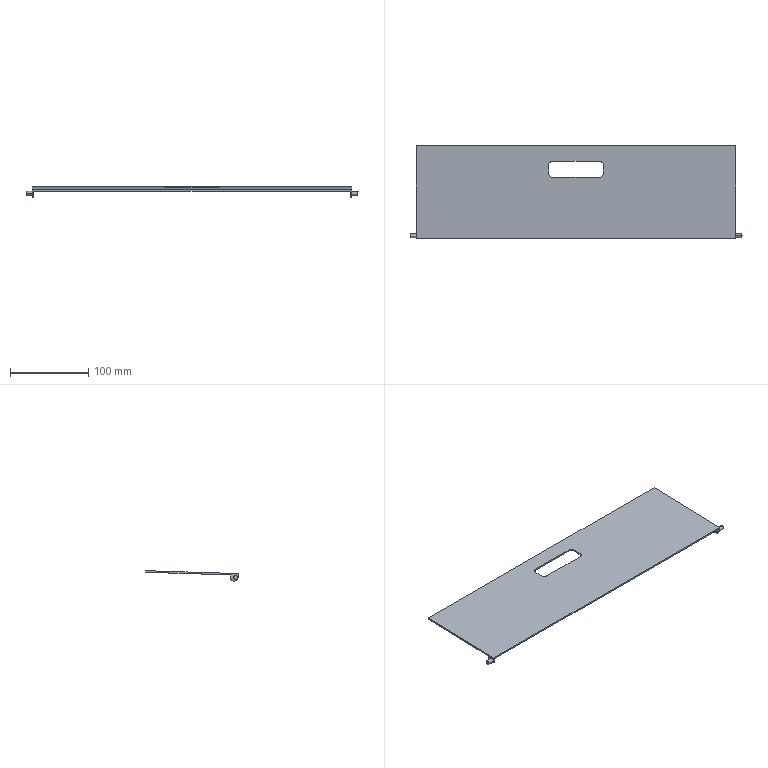Component | SolidWorks | ControlAssembly-1_ControlBoxDoor-1 | 1 solid | 28 faces | box 424 x 118 x 13.61 mm | volume 94122 mm3 | plane 16 | cylinder 12 | commonest cylinder face diameters 10 x8 5 x4
STEP:
#1=COLOUR_RGB('',0.7922,0.8196,0.9333);
#2=FILL_AREA_STYLE_COLOUR('',#1);
#3=FILL_AREA_STYLE('',(#2));
#4=SURFACE_STYLE_FILL_AREA(#3);
#5=SURFACE_SIDE_STYLE('',(#4));
#6=SURFACE_STYLE_USAGE(.BOTH.,#5);
#7=PRESENTATION_STYLE_ASSIGNMENT((#6));
#8=CARTESIAN_POINT('',(14.112,-5.037,19.937));
#9=VERTEX_POINT('',#8);
#10=CARTESIAN_POINT('',(14.112,-4.84,19.943));
#11=VERTEX_POINT('',#10);
#12=CARTESIAN_POINT('',(14.112,-4.938,19.94));
#13=DIRECTION('',(-1.,-0.,0.00009864));
#14=DIRECTION('',(-0.00000312,-0.9995,-0.0316));
#15=AXIS2_PLACEMENT_3D('',#12,#13,#14);
#16=CIRCLE('',#15,0.09843);
#17=EDGE_CURVE('',#9,#11,#16,.T.);
#18=ORIENTED_EDGE('',*,*,#17,.F.);
#19=CARTESIAN_POINT('',(14.427,-5.037,19.937));
#20=VERTEX_POINT('',#19);
#21=CARTESIAN_POINT('',(14.112,-5.037,19.937));
#22=DIRECTION('',(1.,0.,-0.00009864));
#23=VECTOR('',#22,39.37);
#24=LINE('',#21,#23);
#25=EDGE_CURVE('',#9,#20,#24,.T.);
#26=ORIENTED_EDGE('',*,*,#25,.T.);
#27=CARTESIAN_POINT('',(14.427,-4.84,19.943));
#28=VERTEX_POINT('',#27);
#29=CARTESIAN_POINT('',(14.427,-4.938,19.94));
#30=DIRECTION('',(-1.,-0.,0.00009864));
#31=DIRECTION('',(0.00000312,0.9995,0.0316));
#32=AXIS2_PLACEMENT_3D('',#29,#30,#31);
#33=CIRCLE('',#32,0.09843);
#34=EDGE_CURVE('',#20,#28,#33,.T.);
#35=ORIENTED_EDGE('',*,*,#34,.T.);
#36=CARTESIAN_POINT('',(14.112,-4.84,19.943));
#37=DIRECTION('',(1.,0.,-0.00009864));
#38=VECTOR('',#37,39.37);
#39=LINE('',#36,#38);
#40=EDGE_CURVE('',#11,#28,#39,.T.);
#41=ORIENTED_EDGE('',*,*,#40,.F.);
#42=EDGE_LOOP('',(#18,#26,#35,#41));
#43=FACE_OUTER_BOUND('',#42,.T.);
#44=CARTESIAN_POINT('',(14.112,-4.938,19.94));
#45=DIRECTION('',(1.,0.,-0.00009864));
#46=DIRECTION('',(0.00000312,0.9995,0.0316));
#47=AXIS2_PLACEMENT_3D('',#44,#45,#46);
#48=CYLINDRICAL_SURFACE('',#47,0.09843);
#49=ADVANCED_FACE('',(#43),#48,.T.);
#50=CARTESIAN_POINT('',(30.805,-4.935,19.84));
#51=VERTEX_POINT('',#50);
#52=CARTESIAN_POINT('',(30.805,-4.941,20.037));
#53=VERTEX_POINT('',#52);
#54=CARTESIAN_POINT('',(30.805,-4.938,19.938));
#55=DIRECTION('',(1.,-0.,-0.00009864));
#56=DIRECTION('',(-0.00009859,0.0316,-0.9995));
#57=AXIS2_PLACEMENT_3D('',#54,#55,#56);
#58=CIRCLE('',#57,0.09843);
#59=EDGE_CURVE('',#51,#53,#58,.T.);
#60=ORIENTED_EDGE('',*,*,#59,.F.);
#61=CARTESIAN_POINT('',(30.49,-4.935,19.84));
#62=VERTEX_POINT('',#61);
#63=CARTESIAN_POINT('',(30.805,-4.935,19.84));
#64=DIRECTION('',(-1.,0.,0.00009864));
#65=VECTOR('',#64,39.37);
#66=LINE('',#63,#65);
#67=EDGE_CURVE('',#51,#62,#66,.T.);
#68=ORIENTED_EDGE('',*,*,#67,.T.);
#69=CARTESIAN_POINT('',(30.49,-4.941,20.037));
#70=VERTEX_POINT('',#69);
#71=CARTESIAN_POINT('',(30.49,-4.938,19.938));
#72=DIRECTION('',(1.,-0.,-0.00009864));
#73=DIRECTION('',(0.00009859,-0.0316,0.9995));
#74=AXIS2_PLACEMENT_3D('',#71,#72,#73);
#75=CIRCLE('',#74,0.09843);
#76=EDGE_CURVE('',#62,#70,#75,.T.);
#77=ORIENTED_EDGE('',*,*,#76,.T.);
#78=CARTESIAN_POINT('',(30.805,-4.941,20.037));
#79=DIRECTION('',(-1.,0.,0.00009864));
#80=VECTOR('',#79,39.37);
#81=LINE('',#78,#80);
#82=EDGE_CURVE('',#53,#70,#81,.T.);
#83=ORIENTED_EDGE('',*,*,#82,.F.);
#84=EDGE_LOOP('',(#60,#68,#77,#83));
#85=FACE_OUTER_BOUND('',#84,.T.);
#86=CARTESIAN_POINT('',(30.805,-4.938,19.938));
#87=DIRECTION('',(-1.,0.,0.00009864));
#88=DIRECTION('',(0.00009859,-0.0316,0.9995));
#89=AXIS2_PLACEMENT_3D('',#86,#87,#88);
#90=CYLINDRICAL_SURFACE('',#89,0.09843);
#91=ADVANCED_FACE('',(#85),#90,.T.);
#92=CARTESIAN_POINT('',(14.427,-4.663,19.949));
#93=VERTEX_POINT('',#92);
#94=CARTESIAN_POINT('',(14.427,-4.853,19.746));
#95=VERTEX_POINT('',#94);
#96=CARTESIAN_POINT('',(14.427,-4.86,19.942));
#97=DIRECTION('',(-1.,-0.,0.00009864));
#98=DIRECTION('',(0.00000312,0.9995,0.0316));
#99=AXIS2_PLACEMENT_3D('',#96,#97,#98);
#100=CIRCLE('',#99,0.1969);
#101=EDGE_CURVE('',#93,#95,#100,.T.);
#102=ORIENTED_EDGE('',*,*,#101,.T.);
#103=CARTESIAN_POINT('',(14.427,-5.056,19.936));
#104=VERTEX_POINT('',#103);
#105=CARTESIAN_POINT('',(14.427,-4.86,19.942));
#106=DIRECTION('',(-1.,-0.,0.00009864));
#107=DIRECTION('',(0.00000312,0.9995,0.0316));
#108=AXIS2_PLACEMENT_3D('',#105,#106,#107);
#109=CIRCLE('',#108,0.1969);
#110=EDGE_CURVE('',#95,#104,#109,.T.);
#111=ORIENTED_EDGE('',*,*,#110,.T.);
#112=CARTESIAN_POINT('',(14.427,-5.063,20.133));
#113=VERTEX_POINT('',#112);
#114=CARTESIAN_POINT('',(14.427,-5.063,20.133));
#115=DIRECTION('',(-0.00009859,0.0316,-0.9995));
#116=VECTOR('',#115,39.37);
#117=LINE('',#114,#116);
#118=EDGE_CURVE('',#113,#104,#117,.T.);
#119=ORIENTED_EDGE('',*,*,#118,.F.);
#120=CARTESIAN_POINT('',(14.427,-0.4193,20.28));
#121=VERTEX_POINT('',#120);
#122=CARTESIAN_POINT('',(14.427,-0.4193,20.28));
#123=DIRECTION('',(-0.00000312,-0.9995,-0.0316));
#124=VECTOR('',#123,39.37);
#125=LINE('',#122,#124);
#126=EDGE_CURVE('',#121,#113,#125,.T.);
#127=ORIENTED_EDGE('',*,*,#126,.F.);
#128=CARTESIAN_POINT('',(14.427,-0.4168,20.201));
#129=VERTEX_POINT('',#128);
#130=CARTESIAN_POINT('',(14.427,-0.4193,20.28));
#131=DIRECTION('',(-0.00009859,0.0316,-0.9995));
#132=VECTOR('',#131,39.37);
#133=LINE('',#130,#132);
#134=EDGE_CURVE('',#121,#129,#133,.T.);
#135=ORIENTED_EDGE('',*,*,#134,.T.);
#136=CARTESIAN_POINT('',(14.427,-4.667,20.067));
#137=VERTEX_POINT('',#136);
#138=CARTESIAN_POINT('',(14.427,-0.4168,20.201));
#139=DIRECTION('',(-0.00000312,-0.9995,-0.0316));
#140=VECTOR('',#139,39.37);
#141=LINE('',#138,#140);
#142=EDGE_CURVE('',#129,#137,#141,.T.);
#143=ORIENTED_EDGE('',*,*,#142,.T.);
#144=CARTESIAN_POINT('',(14.427,-4.669,20.145));
#145=DIRECTION('',(-0.00009859,0.0316,-0.9995));
#146=VECTOR('',#145,39.37);
#147=LINE('',#144,#146);
#148=EDGE_CURVE('',#137,#93,#147,.T.);
#149=ORIENTED_EDGE('',*,*,#148,.T.);
#150=EDGE_LOOP('',(#102,#111,#119,#127,#135,#143,#149));
#151=FACE_OUTER_BOUND('',#150,.T.);
#152=CARTESIAN_POINT('',(14.427,-4.938,19.94));
#153=DIRECTION('',(-1.,-0.,0.00009864));
#154=DIRECTION('',(0.00000312,0.9995,0.0316));
#155=AXIS2_PLACEMENT_3D('',#152,#153,#154);
#156=CIRCLE('',#155,0.09843);
#157=EDGE_CURVE('',#28,#20,#156,.T.);
#158=ORIENTED_EDGE('',*,*,#157,.F.);
#159=ORIENTED_EDGE('',*,*,#34,.F.);
#160=EDGE_LOOP('',(#158,#159));
#161=FACE_BOUND('',#160,.T.);
#162=CARTESIAN_POINT('',(14.427,-0.4193,20.28));
#163=DIRECTION('',(1.,0.,-0.00009864));
#164=DIRECTION('',(0.00000312,0.9995,0.0316));
#165=AXIS2_PLACEMENT_3D('',#162,#163,#164);
#166=PLANE('',#165);
#167=ADVANCED_FACE('',(#151,#161),#166,.F.);
#168=CARTESIAN_POINT('',(30.49,-5.063,20.131));
#169=VERTEX_POINT('',#168);
#170=CARTESIAN_POINT('',(30.49,-5.056,19.935));
#171=VERTEX_POINT('',#170);
#172=CARTESIAN_POINT('',(30.49,-5.063,20.131));
#173=DIRECTION('',(-0.00009859,0.0316,-0.9995));
#174=VECTOR('',#173,39.37);
#175=LINE('',#172,#174);
#176=EDGE_CURVE('',#169,#171,#175,.T.);
#177=ORIENTED_EDGE('',*,*,#176,.T.);
#178=CARTESIAN_POINT('',(30.49,-4.853,19.744));
#179=VERTEX_POINT('',#178);
#180=CARTESIAN_POINT('',(30.49,-4.86,19.941));
#181=DIRECTION('',(1.,-0.,-0.00009864));
#182=DIRECTION('',(0.00009859,-0.0316,0.9995));
#183=AXIS2_PLACEMENT_3D('',#180,#181,#182);
#184=CIRCLE('',#183,0.1969);
#185=EDGE_CURVE('',#171,#179,#184,.T.);
#186=ORIENTED_EDGE('',*,*,#185,.T.);
#187=CARTESIAN_POINT('',(30.49,-4.663,19.947));
#188=VERTEX_POINT('',#187);
#189=CARTESIAN_POINT('',(30.49,-4.86,19.941));
#190=DIRECTION('',(1.,-0.,-0.00009864));
#191=DIRECTION('',(0.00009859,-0.0316,0.9995));
#192=AXIS2_PLACEMENT_3D('',#189,#190,#191);
#193=CIRCLE('',#192,0.1969);
#194=EDGE_CURVE('',#179,#188,#193,.T.);
#195=ORIENTED_EDGE('',*,*,#194,.T.);
#196=CARTESIAN_POINT('',(30.49,-4.667,20.065));
#197=VERTEX_POINT('',#196);
#198=CARTESIAN_POINT('',(30.49,-4.669,20.144));
#199=DIRECTION('',(0.00009859,-0.0316,0.9995));
#200=VECTOR('',#199,39.37);
#201=LINE('',#198,#200);
#202=EDGE_CURVE('',#188,#197,#201,.T.);
#203=ORIENTED_EDGE('',*,*,#202,.T.);
#204=CARTESIAN_POINT('',(30.49,-0.4168,20.2));
#205=VERTEX_POINT('',#204);
#206=CARTESIAN_POINT('',(30.49,-0.4168,20.2));
#207=DIRECTION('',(0.00000312,0.9995,0.0316));
#208=VECTOR('',#207,39.37);
#209=LINE('',#206,#208);
#210=EDGE_CURVE('',#197,#205,#209,.T.);
#211=ORIENTED_EDGE('',*,*,#210,.T.);
#212=CARTESIAN_POINT('',(30.49,-0.4193,20.278));
#213=VERTEX_POINT('',#212);
#214=CARTESIAN_POINT('',(30.49,-0.4193,20.278));
#215=DIRECTION('',(-0.00009859,0.0316,-0.9995));
#216=VECTOR('',#215,39.37);
#217=LINE('',#214,#216);
#218=EDGE_CURVE('',#213,#205,#217,.T.);
#219=ORIENTED_EDGE('',*,*,#218,.F.);
#220=CARTESIAN_POINT('',(30.49,-0.4193,20.278));
#221=DIRECTION('',(0.00000312,0.9995,0.0316));
#222=VECTOR('',#221,39.37);
#223=LINE('',#220,#222);
#224=EDGE_CURVE('',#169,#213,#223,.T.);
#225=ORIENTED_EDGE('',*,*,#224,.F.);
#226=EDGE_LOOP('',(#177,#186,#195,#203,#211,#219,#225));
#227=FACE_OUTER_BOUND('',#226,.T.);
#228=CARTESIAN_POINT('',(30.49,-4.938,19.938));
#229=DIRECTION('',(1.,-0.,-0.00009864));
#230=DIRECTION('',(0.00009859,-0.0316,0.9995));
#231=AXIS2_PLACEMENT_3D('',#228,#229,#230);
#232=CIRCLE('',#231,0.09843);
#233=EDGE_CURVE('',#70,#62,#232,.T.);
#234=ORIENTED_EDGE('',*,*,#233,.F.);
#235=ORIENTED_EDGE('',*,*,#76,.F.);
#236=EDGE_LOOP('',(#234,#235));
#237=FACE_BOUND('',#236,.T.);
#238=CARTESIAN_POINT('',(30.49,-0.4193,20.278));
#239=DIRECTION('',(-1.,0.,0.00009864));
#240=DIRECTION('',(0.00009859,-0.0316,0.9995));
#241=AXIS2_PLACEMENT_3D('',#238,#239,#240);
#242=PLANE('',#241);
#243=ADVANCED_FACE('',(#227,#237),#242,.F.);
#244=ORIENTED_EDGE('',*,*,#118,.T.);
#245=CARTESIAN_POINT('',(14.506,-5.056,19.936));
#246=VERTEX_POINT('',#245);
#247=CARTESIAN_POINT('',(14.506,-5.056,19.936));
#248=DIRECTION('',(1.,-0.,-0.00009864));
#249=VECTOR('',#248,39.37);
#250=LINE('',#247,#249);
#251=EDGE_CURVE('',#104,#246,#250,.T.);
#252=ORIENTED_EDGE('',*,*,#251,.T.);
#253=CARTESIAN_POINT('',(14.506,-5.06,20.054));
#254=VERTEX_POINT('',#253);
#255=CARTESIAN_POINT('',(14.506,-5.063,20.133));
#256=DIRECTION('',(0.00009859,-0.0316,0.9995));
#257=VECTOR('',#256,39.37);
#258=LINE('',#255,#257);
#259=EDGE_CURVE('',#246,#254,#258,.T.);
#260=ORIENTED_EDGE('',*,*,#259,.T.);
#261=CARTESIAN_POINT('',(30.412,-5.06,20.053));
#262=VERTEX_POINT('',#261);
#263=CARTESIAN_POINT('',(14.427,-5.06,20.054));
#264=DIRECTION('',(1.,-0.,-0.00009864));
#265=VECTOR('',#264,39.37);
#266=LINE('',#263,#265);
#267=EDGE_CURVE('',#254,#262,#266,.T.);
#268=ORIENTED_EDGE('',*,*,#267,.T.);
#269=CARTESIAN_POINT('',(30.412,-5.056,19.935));
#270=VERTEX_POINT('',#269);
#271=CARTESIAN_POINT('',(30.412,-5.063,20.131));
#272=DIRECTION('',(-0.00009859,0.0316,-0.9995));
#273=VECTOR('',#272,39.37);
#274=LINE('',#271,#273);
#275=EDGE_CURVE('',#262,#270,#274,.T.);
#276=ORIENTED_EDGE('',*,*,#275,.T.);
#277=CARTESIAN_POINT('',(30.49,-5.056,19.935));
#278=DIRECTION('',(1.,-0.,-0.00009864));
#279=VECTOR('',#278,39.37);
#280=LINE('',#277,#279);
#281=EDGE_CURVE('',#270,#171,#280,.T.);
#282=ORIENTED_EDGE('',*,*,#281,.T.);
#283=ORIENTED_EDGE('',*,*,#176,.F.);
#284=CARTESIAN_POINT('',(14.427,-5.063,20.133));
#285=DIRECTION('',(1.,-0.,-0.00009864));
#286=VECTOR('',#285,39.37);
#287=LINE('',#284,#286);
#288=EDGE_CURVE('',#113,#169,#287,.T.);
#289=ORIENTED_EDGE('',*,*,#288,.F.);
#290=EDGE_LOOP('',(#244,#252,#260,#268,#276,#282,#283,#289));
#291=FACE_OUTER_BOUND('',#290,.T.);
#292=CARTESIAN_POINT('',(14.427,-5.063,20.133));
#293=DIRECTION('',(0.00000312,0.9995,0.0316));
#294=DIRECTION('',(0.00009859,-0.0316,0.9995));
#295=AXIS2_PLACEMENT_3D('',#292,#293,#294);
#296=PLANE('',#295);
#297=ADVANCED_FACE('',(#291),#296,.F.);
#298=CARTESIAN_POINT('',(14.427,-0.4168,20.201));
#299=DIRECTION('',(-1.,0.,0.00009864));
#300=VECTOR('',#299,39.37);
#301=LINE('',#298,#300);
#302=EDGE_CURVE('',#205,#129,#301,.T.);
#303=ORIENTED_EDGE('',*,*,#302,.T.);
#304=ORIENTED_EDGE('',*,*,#134,.F.);
#305=CARTESIAN_POINT('',(14.427,-0.4193,20.28));
#306=DIRECTION('',(-1.,0.,0.00009864));
#307=VECTOR('',#306,39.37);
#308=LINE('',#305,#307);
#309=EDGE_CURVE('',#213,#121,#308,.T.);
#310=ORIENTED_EDGE('',*,*,#309,.F.);
#311=ORIENTED_EDGE('',*,*,#218,.T.);
#312=EDGE_LOOP('',(#303,#304,#310,#311));
#313=FACE_OUTER_BOUND('',#312,.T.);
#314=CARTESIAN_POINT('',(14.427,-0.4193,20.28));
#315=DIRECTION('',(-0.00000312,-0.9995,-0.0316));
#316=DIRECTION('',(-0.00009859,0.0316,-0.9995));
#317=AXIS2_PLACEMENT_3D('',#314,#315,#316);
#318=PLANE('',#317);
#319=ADVANCED_FACE('',(#313),#318,.F.);
#320=CARTESIAN_POINT('',(21.081,-1.403,20.248));
#321=VERTEX_POINT('',#320);
#322=CARTESIAN_POINT('',(21.081,-1.797,20.236));
#323=VERTEX_POINT('',#322);
#324=CARTESIAN_POINT('',(21.081,-1.206,20.254));
#325=DIRECTION('',(-0.00000312,-0.9995,-0.0316));
#326=VECTOR('',#325,39.37);
#327=LINE('',#324,#326);
#328=EDGE_CURVE('',#321,#323,#327,.T.);
#329=ORIENTED_EDGE('',*,*,#328,.F.);
#330=CARTESIAN_POINT('',(21.278,-1.206,20.254));
#331=VERTEX_POINT('',#330);
#332=CARTESIAN_POINT('',(21.278,-1.403,20.248));
#333=DIRECTION('',(-0.00009859,0.0316,-0.9995));
#334=DIRECTION('',(1.,0.,-0.00009864));
#335=AXIS2_PLACEMENT_3D('',#332,#333,#334);
#336=CIRCLE('',#335,0.1969);
#337=EDGE_CURVE('',#321,#331,#336,.T.);
#338=ORIENTED_EDGE('',*,*,#337,.T.);
#339=CARTESIAN_POINT('',(23.64,-1.206,20.254));
#340=VERTEX_POINT('',#339);
#341=CARTESIAN_POINT('',(21.081,-1.206,20.254));
#342=DIRECTION('',(-1.,0.,0.00009864));
#343=VECTOR('',#342,39.37);
#344=LINE('',#341,#343);
#345=EDGE_CURVE('',#340,#331,#344,.T.);
#346=ORIENTED_EDGE('',*,*,#345,.F.);
#347=CARTESIAN_POINT('',(23.837,-1.403,20.248));
#348=VERTEX_POINT('',#347);
#349=CARTESIAN_POINT('',(23.64,-1.403,20.248));
#350=DIRECTION('',(-0.00009859,0.0316,-0.9995));
#351=DIRECTION('',(1.,-0.,-0.00009864));
#352=AXIS2_PLACEMENT_3D('',#349,#350,#351);
#353=CIRCLE('',#352,0.1969);
#354=EDGE_CURVE('',#340,#348,#353,.T.);
#355=ORIENTED_EDGE('',*,*,#354,.T.);
#356=CARTESIAN_POINT('',(23.837,-1.797,20.235));
#357=VERTEX_POINT('',#356);
#358=CARTESIAN_POINT('',(23.837,-1.206,20.254));
#359=DIRECTION('',(0.00000312,0.9995,0.0316));
#360=VECTOR('',#359,39.37);
#361=LINE('',#358,#360);
#362=EDGE_CURVE('',#357,#348,#361,.T.);
#363=ORIENTED_EDGE('',*,*,#362,.F.);
#364=CARTESIAN_POINT('',(23.64,-1.993,20.229));
#365=VERTEX_POINT('',#364);
#366=CARTESIAN_POINT('',(23.64,-1.797,20.235));
#367=DIRECTION('',(-0.00009859,0.0316,-0.9995));
#368=DIRECTION('',(1.,0.,-0.00009864));
#369=AXIS2_PLACEMENT_3D('',#366,#367,#368);
#370=CIRCLE('',#369,0.1969);
#371=EDGE_CURVE('',#357,#365,#370,.T.);
#372=ORIENTED_EDGE('',*,*,#371,.T.);
#373=CARTESIAN_POINT('',(21.278,-1.993,20.229));
#374=VERTEX_POINT('',#373);
#375=CARTESIAN_POINT('',(21.081,-1.993,20.229));
#376=DIRECTION('',(1.,-0.,-0.00009864));
#377=VECTOR('',#376,39.37);
#378=LINE('',#375,#377);
#379=EDGE_CURVE('',#374,#365,#378,.T.);
#380=ORIENTED_EDGE('',*,*,#379,.F.);
#381=CARTESIAN_POINT('',(21.278,-1.797,20.236));
#382=DIRECTION('',(-0.00009859,0.0316,-0.9995));
#383=DIRECTION('',(1.,0.,-0.00009864));
#384=AXIS2_PLACEMENT_3D('',#381,#382,#383);
#385=CIRCLE('',#384,0.1969);
#386=EDGE_CURVE('',#374,#323,#385,.T.);
#387=ORIENTED_EDGE('',*,*,#386,.T.);
#388=EDGE_LOOP('',(#329,#338,#346,#355,#363,#372,#380,#387));
#389=FACE_BOUND('',#388,.T.);
#390=ORIENTED_EDGE('',*,*,#126,.T.);
#391=ORIENTED_EDGE('',*,*,#288,.T.);
#392=ORIENTED_EDGE('',*,*,#224,.T.);
#393=ORIENTED_EDGE('',*,*,#309,.T.);
#394=EDGE_LOOP('',(#390,#391,#392,#393));
#395=FACE_OUTER_BOUND('',#394,.T.);
#396=CARTESIAN_POINT('',(17.068,-0.9992,20.261));
#397=DIRECTION('',(0.00009859,-0.0316,0.9995));
#398=DIRECTION('',(1.,-0.,-0.00009864));
#399=AXIS2_PLACEMENT_3D('',#396,#397,#398);
#400=PLANE('',#399);
#401=ADVANCED_FACE('',(#389,#395),#400,.T.);
#402=CARTESIAN_POINT('',(23.837,-1.794,20.157));
#403=VERTEX_POINT('',#402);
#404=CARTESIAN_POINT('',(23.837,-1.401,20.169));
#405=VERTEX_POINT('',#404);
#406=CARTESIAN_POINT('',(23.837,-1.204,20.175));
#407=DIRECTION('',(0.00000312,0.9995,0.0316));
#408=VECTOR('',#407,39.37);
#409=LINE('',#406,#408);
#410=EDGE_CURVE('',#403,#405,#409,.T.);
#411=ORIENTED_EDGE('',*,*,#410,.T.);
#412=CARTESIAN_POINT('',(23.64,-1.204,20.175));
#413=VERTEX_POINT('',#412);
#414=CARTESIAN_POINT('',(23.64,-1.401,20.169));
#415=DIRECTION('',(0.00009859,-0.0316,0.9995));
#416=DIRECTION('',(1.,0.,-0.00009864));
#417=AXIS2_PLACEMENT_3D('',#414,#415,#416);
#418=CIRCLE('',#417,0.1969);
#419=EDGE_CURVE('',#405,#413,#418,.T.);
#420=ORIENTED_EDGE('',*,*,#419,.T.);
#421=CARTESIAN_POINT('',(21.278,-1.204,20.176));
#422=VERTEX_POINT('',#421);
#423=CARTESIAN_POINT('',(21.081,-1.204,20.176));
#424=DIRECTION('',(-1.,0.,0.00009864));
#425=VECTOR('',#424,39.37);
#426=LINE('',#423,#425);
#427=EDGE_CURVE('',#413,#422,#426,.T.);
#428=ORIENTED_EDGE('',*,*,#427,.T.);
#429=CARTESIAN_POINT('',(21.081,-1.401,20.169));
#430=VERTEX_POINT('',#429);
#431=CARTESIAN_POINT('',(21.278,-1.401,20.169));
#432=DIRECTION('',(0.00009859,-0.0316,0.9995));
#433=DIRECTION('',(1.,0.,-0.00009864));
#434=AXIS2_PLACEMENT_3D('',#431,#432,#433);
#435=CIRCLE('',#434,0.1969);
#436=EDGE_CURVE('',#422,#430,#435,.T.);
#437=ORIENTED_EDGE('',*,*,#436,.T.);
#438=CARTESIAN_POINT('',(21.081,-1.794,20.157));
#439=VERTEX_POINT('',#438);
#440=CARTESIAN_POINT('',(21.081,-1.204,20.176));
#441=DIRECTION('',(-0.00000312,-0.9995,-0.0316));
#442=VECTOR('',#441,39.37);
#443=LINE('',#440,#442);
#444=EDGE_CURVE('',#430,#439,#443,.T.);
#445=ORIENTED_EDGE('',*,*,#444,.T.);
#446=CARTESIAN_POINT('',(21.278,-1.991,20.151));
#447=VERTEX_POINT('',#446);
#448=CARTESIAN_POINT('',(21.278,-1.794,20.157));
#449=DIRECTION('',(0.00009859,-0.0316,0.9995));
#450=DIRECTION('',(1.,0.,-0.00009864));
#451=AXIS2_PLACEMENT_3D('',#448,#449,#450);
#452=CIRCLE('',#451,0.1969);
#453=EDGE_CURVE('',#439,#447,#452,.T.);
#454=ORIENTED_EDGE('',*,*,#453,.T.);
#455=CARTESIAN_POINT('',(23.64,-1.991,20.15));
#456=VERTEX_POINT('',#455);
#457=CARTESIAN_POINT('',(21.081,-1.991,20.151));
#458=DIRECTION('',(1.,-0.,-0.00009864));
#459=VECTOR('',#458,39.37);
#460=LINE('',#457,#459);
#461=EDGE_CURVE('',#447,#456,#460,.T.);
#462=ORIENTED_EDGE('',*,*,#461,.T.);
#463=CARTESIAN_POINT('',(23.64,-1.794,20.157));
#464=DIRECTION('',(0.00009859,-0.0316,0.9995));
#465=DIRECTION('',(1.,0.,-0.00009864));
#466=AXIS2_PLACEMENT_3D('',#463,#464,#465);
#467=CIRCLE('',#466,0.1969);
#468=EDGE_CURVE('',#456,#403,#467,.T.);
#469=ORIENTED_EDGE('',*,*,#468,.T.);
#470=EDGE_LOOP('',(#411,#420,#428,#437,#445,#454,#462,#469));
#471=FACE_BOUND('',#470,.T.);
#472=CARTESIAN_POINT('',(14.506,-4.667,20.067));
#473=VERTEX_POINT('',#472);
#474=CARTESIAN_POINT('',(14.506,-0.9967,20.183));
#475=DIRECTION('',(-0.00000312,-0.9995,-0.0316));
#476=VECTOR('',#475,39.37);
#477=LINE('',#474,#476);
#478=EDGE_CURVE('',#473,#254,#477,.T.);
#479=ORIENTED_EDGE('',*,*,#478,.F.);
#480=CARTESIAN_POINT('',(17.068,-4.667,20.066));
#481=DIRECTION('',(-1.,-0.,0.00009864));
#482=VECTOR('',#481,39.37);
#483=LINE('',#480,#482);
#484=EDGE_CURVE('',#473,#137,#483,.T.);
#485=ORIENTED_EDGE('',*,*,#484,.T.);
#486=ORIENTED_EDGE('',*,*,#142,.F.);
#487=ORIENTED_EDGE('',*,*,#302,.F.);
#488=ORIENTED_EDGE('',*,*,#210,.F.);
#489=CARTESIAN_POINT('',(30.412,-4.667,20.065));
#490=VERTEX_POINT('',#489);
#491=CARTESIAN_POINT('',(17.068,-4.667,20.066));
#492=DIRECTION('',(-1.,0.,0.00009864));
#493=VECTOR('',#492,39.37);
#494=LINE('',#491,#493);
#495=EDGE_CURVE('',#197,#490,#494,.T.);
#496=ORIENTED_EDGE('',*,*,#495,.T.);
#497=CARTESIAN_POINT('',(30.412,-0.9967,20.181));
#498=DIRECTION('',(0.00000312,0.9995,0.0316));
#499=VECTOR('',#498,39.37);
#500=LINE('',#497,#499);
#501=EDGE_CURVE('',#262,#490,#500,.T.);
#502=ORIENTED_EDGE('',*,*,#501,.F.);
#503=ORIENTED_EDGE('',*,*,#267,.F.);
#504=EDGE_LOOP('',(#479,#485,#486,#487,#488,#496,#502,#503));
#505=FACE_OUTER_BOUND('',#504,.T.);
#506=CARTESIAN_POINT('',(17.068,-0.9967,20.182));
#507=DIRECTION('',(0.00009859,-0.0316,0.9995));
#508=DIRECTION('',(1.,-0.,-0.00009864));
#509=AXIS2_PLACEMENT_3D('',#506,#507,#508);
#510=PLANE('',#509);
#511=ADVANCED_FACE('',(#471,#505),#510,.F.);
#512=ORIENTED_EDGE('',*,*,#202,.F.);
#513=CARTESIAN_POINT('',(30.412,-4.663,19.947));
#514=VERTEX_POINT('',#513);
#515=CARTESIAN_POINT('',(30.412,-4.663,19.947));
#516=DIRECTION('',(-1.,0.,0.00009864));
#517=VECTOR('',#516,39.37);
#518=LINE('',#515,#517);
#519=EDGE_CURVE('',#188,#514,#518,.T.);
#520=ORIENTED_EDGE('',*,*,#519,.T.);
#521=CARTESIAN_POINT('',(30.412,-4.669,20.144));
#522=DIRECTION('',(0.00009859,-0.0316,0.9995));
#523=VECTOR('',#522,39.37);
#524=LINE('',#521,#523);
#525=EDGE_CURVE('',#514,#490,#524,.T.);
#526=ORIENTED_EDGE('',*,*,#525,.T.);
#527=ORIENTED_EDGE('',*,*,#495,.F.);
#528=EDGE_LOOP('',(#512,#520,#526,#527));
#529=FACE_OUTER_BOUND('',#528,.T.);
#530=CARTESIAN_POINT('',(30.412,-4.669,20.144));
#531=DIRECTION('',(0.00000312,0.9995,0.0316));
#532=DIRECTION('',(0.00009859,-0.0316,0.9995));
#533=AXIS2_PLACEMENT_3D('',#530,#531,#532);
#534=PLANE('',#533);
#535=ADVANCED_FACE('',(#529),#534,.T.);
#536=CARTESIAN_POINT('',(30.412,-4.853,19.744));
#537=VERTEX_POINT('',#536);
#538=CARTESIAN_POINT('',(30.412,-4.86,19.941));
#539=DIRECTION('',(-1.,0.,0.00009864));
#540=DIRECTION('',(-0.00009859,0.0316,-0.9995));
#541=AXIS2_PLACEMENT_3D('',#538,#539,#540);
#542=CIRCLE('',#541,0.1969);
#543=EDGE_CURVE('',#514,#537,#542,.T.);
#544=ORIENTED_EDGE('',*,*,#543,.T.);
#545=CARTESIAN_POINT('',(30.412,-4.86,19.941));
#546=DIRECTION('',(-1.,0.,0.00009864));
#547=DIRECTION('',(-0.00009859,0.0316,-0.9995));
#548=AXIS2_PLACEMENT_3D('',#545,#546,#547);
#549=CIRCLE('',#548,0.1969);
#550=EDGE_CURVE('',#537,#270,#549,.T.);
#551=ORIENTED_EDGE('',*,*,#550,.T.);
#552=ORIENTED_EDGE('',*,*,#275,.F.);
#553=ORIENTED_EDGE('',*,*,#501,.T.);
#554=ORIENTED_EDGE('',*,*,#525,.F.);
#555=EDGE_LOOP('',(#544,#551,#552,#553,#554));
#556=FACE_OUTER_BOUND('',#555,.T.);
#557=CARTESIAN_POINT('',(30.412,-0.9967,20.181));
#558=DIRECTION('',(1.,-0.,-0.00009864));
#559=DIRECTION('',(-0.00009859,0.0316,-0.9995));
#560=AXIS2_PLACEMENT_3D('',#557,#558,#559);
#561=PLANE('',#560);
#562=ADVANCED_FACE('',(#556),#561,.F.);
#563=CARTESIAN_POINT('',(14.506,-4.663,19.949));
#564=VERTEX_POINT('',#563);
#565=CARTESIAN_POINT('',(14.506,-4.669,20.145));
#566=DIRECTION('',(-0.00009859,0.0316,-0.9995));
#567=VECTOR('',#566,39.37);
#568=LINE('',#565,#567);
#569=EDGE_CURVE('',#473,#564,#568,.T.);
#570=ORIENTED_EDGE('',*,*,#569,.T.);
#571=CARTESIAN_POINT('',(14.506,-4.663,19.949));
#572=DIRECTION('',(-1.,-0.,0.00009864));
#573=VECTOR('',#572,39.37);
#574=LINE('',#571,#573);
#575=EDGE_CURVE('',#564,#93,#574,.T.);
#576=ORIENTED_EDGE('',*,*,#575,.T.);
#577=ORIENTED_EDGE('',*,*,#148,.F.);
#578=ORIENTED_EDGE('',*,*,#484,.F.);
#579=EDGE_LOOP('',(#570,#576,#577,#578));
#580=FACE_OUTER_BOUND('',#579,.T.);
#581=CARTESIAN_POINT('',(14.506,-4.669,20.145));
#582=DIRECTION('',(0.00000312,0.9995,0.0316));
#583=DIRECTION('',(0.00009859,-0.0316,0.9995));
#584=AXIS2_PLACEMENT_3D('',#581,#582,#583);
#585=PLANE('',#584);
#586=ADVANCED_FACE('',(#580),#585,.T.);
#587=ORIENTED_EDGE('',*,*,#259,.F.);
#588=CARTESIAN_POINT('',(14.506,-4.853,19.746));
#589=VERTEX_POINT('',#588);
#590=CARTESIAN_POINT('',(14.506,-4.86,19.942));
#591=DIRECTION('',(1.,-0.,-0.00009864));
#592=DIRECTION('',(0.00009859,-0.0316,0.9995));
#593=AXIS2_PLACEMENT_3D('',#590,#591,#592);
#594=CIRCLE('',#593,0.1969);
#595=EDGE_CURVE('',#246,#589,#594,.T.);
#596=ORIENTED_EDGE('',*,*,#595,.T.);
#597=CARTESIAN_POINT('',(14.506,-4.86,19.942));
#598=DIRECTION('',(1.,-0.,-0.00009864));
#599=DIRECTION('',(0.00009859,-0.0316,0.9995));
#600=AXIS2_PLACEMENT_3D('',#597,#598,#599);
#601=CIRCLE('',#600,0.1969);
#602=EDGE_CURVE('',#589,#564,#601,.T.);
#603=ORIENTED_EDGE('',*,*,#602,.T.);
#604=ORIENTED_EDGE('',*,*,#569,.F.);
#605=ORIENTED_EDGE('',*,*,#478,.T.);
#606=EDGE_LOOP('',(#587,#596,#603,#604,#605));
#607=FACE_OUTER_BOUND('',#606,.T.);
#608=CARTESIAN_POINT('',(14.506,-0.9967,20.183));
#609=DIRECTION('',(-1.,0.,0.00009864));
#610=DIRECTION('',(0.00009859,-0.0316,0.9995));
#611=AXIS2_PLACEMENT_3D('',#608,#609,#610);
#612=PLANE('',#611);
#613=ADVANCED_FACE('',(#607),#612,.F.);
#614=ORIENTED_EDGE('',*,*,#328,.T.);
#615=CARTESIAN_POINT('',(21.081,-1.794,20.157));
#616=DIRECTION('',(-0.00009859,0.0316,-0.9995));
#617=VECTOR('',#616,39.37);
#618=LINE('',#615,#617);
#619=EDGE_CURVE('',#323,#439,#618,.T.);
#620=ORIENTED_EDGE('',*,*,#619,.T.);
#621=ORIENTED_EDGE('',*,*,#444,.F.);
#622=CARTESIAN_POINT('',(21.081,-1.403,20.248));
#623=DIRECTION('',(0.00009859,-0.0316,0.9995));
#624=VECTOR('',#623,39.37);
#625=LINE('',#622,#624);
#626=EDGE_CURVE('',#430,#321,#625,.T.);
#627=ORIENTED_EDGE('',*,*,#626,.T.);
#628=EDGE_LOOP('',(#614,#620,#621,#627));
#629=FACE_OUTER_BOUND('',#628,.T.);
#630=CARTESIAN_POINT('',(21.081,-1.204,20.176));
#631=DIRECTION('',(-1.,0.,0.00009864));
#632=DIRECTION('',(0.00009859,-0.0316,0.9995));
#633=AXIS2_PLACEMENT_3D('',#630,#631,#632);
#634=PLANE('',#633);
#635=ADVANCED_FACE('',(#629),#634,.F.);
#636=ORIENTED_EDGE('',*,*,#427,.F.);
#637=CARTESIAN_POINT('',(23.64,-1.206,20.254));
#638=DIRECTION('',(0.00009859,-0.0316,0.9995));
#639=VECTOR('',#638,39.37);
#640=LINE('',#637,#639);
#641=EDGE_CURVE('',#413,#340,#640,.T.);
#642=ORIENTED_EDGE('',*,*,#641,.T.);
#643=ORIENTED_EDGE('',*,*,#345,.T.);
#644=CARTESIAN_POINT('',(21.278,-1.204,20.176));
#645=DIRECTION('',(-0.00009859,0.0316,-0.9995));
#646=VECTOR('',#645,39.37);
#647=LINE('',#644,#646);
#648=EDGE_CURVE('',#331,#422,#647,.T.);
#649=ORIENTED_EDGE('',*,*,#648,.T.);
#650=EDGE_LOOP('',(#636,#642,#643,#649));
#651=FACE_OUTER_BOUND('',#650,.T.);
#652=CARTESIAN_POINT('',(21.081,-1.204,20.176));
#653=DIRECTION('',(0.00000312,0.9995,0.0316));
#654=DIRECTION('',(0.00009859,-0.0316,0.9995));
#655=AXIS2_PLACEMENT_3D('',#652,#653,#654);
#656=PLANE('',#655);
#657=ADVANCED_FACE('',(#651),#656,.F.);
#658=ORIENTED_EDGE('',*,*,#362,.T.);
#659=CARTESIAN_POINT('',(23.837,-1.401,20.169));
#660=DIRECTION('',(-0.00009859,0.0316,-0.9995));
#661=VECTOR('',#660,39.37);
#662=LINE('',#659,#661);
#663=EDGE_CURVE('',#348,#405,#662,.T.);
#664=ORIENTED_EDGE('',*,*,#663,.T.);
#665=ORIENTED_EDGE('',*,*,#410,.F.);
#666=CARTESIAN_POINT('',(23.837,-1.797,20.235));
#667=DIRECTION('',(0.00009859,-0.0316,0.9995));
#668=VECTOR('',#667,39.37);
#669=LINE('',#666,#668);
#670=EDGE_CURVE('',#403,#357,#669,.T.);
#671=ORIENTED_EDGE('',*,*,#670,.T.);
#672=EDGE_LOOP('',(#658,#664,#665,#671));
#673=FACE_OUTER_BOUND('',#672,.T.);
#674=CARTESIAN_POINT('',(23.837,-1.204,20.175));
#675=DIRECTION('',(1.,-0.,-0.00009864));
#676=DIRECTION('',(-0.00009859,0.0316,-0.9995));
#677=AXIS2_PLACEMENT_3D('',#674,#675,#676);
#678=PLANE('',#677);
#679=ADVANCED_FACE('',(#673),#678,.F.);
#680=ORIENTED_EDGE('',*,*,#379,.T.);
#681=CARTESIAN_POINT('',(23.64,-1.991,20.15));
#682=DIRECTION('',(-0.00009859,0.0316,-0.9995));
#683=VECTOR('',#682,39.37);
#684=LINE('',#681,#683);
#685=EDGE_CURVE('',#365,#456,#684,.T.);
#686=ORIENTED_EDGE('',*,*,#685,.T.);
#687=ORIENTED_EDGE('',*,*,#461,.F.);
#688=CARTESIAN_POINT('',(21.278,-1.993,20.229));
#689=DIRECTION('',(0.00009859,-0.0316,0.9995));
#690=VECTOR('',#689,39.37);
#691=LINE('',#688,#690);
#692=EDGE_CURVE('',#447,#374,#691,.T.);
#693=ORIENTED_EDGE('',*,*,#692,.T.);
#694=EDGE_LOOP('',(#680,#686,#687,#693));
#695=FACE_OUTER_BOUND('',#694,.T.);
#696=CARTESIAN_POINT('',(21.081,-1.991,20.151));
#697=DIRECTION('',(-0.00000312,-0.9995,-0.0316));
#698=DIRECTION('',(-0.00009859,0.0316,-0.9995));
#699=AXIS2_PLACEMENT_3D('',#696,#697,#698);
#700=PLANE('',#699);
#701=ADVANCED_FACE('',(#695),#700,.F.);
#702=ORIENTED_EDGE('',*,*,#575,.F.);
#703=ORIENTED_EDGE('',*,*,#602,.F.);
#704=CARTESIAN_POINT('',(14.506,-4.853,19.746));
#705=DIRECTION('',(1.,0.,-0.00009864));
#706=VECTOR('',#705,39.37);
#707=LINE('',#704,#706);
#708=EDGE_CURVE('',#95,#589,#707,.T.);
#709=ORIENTED_EDGE('',*,*,#708,.F.);
#710=ORIENTED_EDGE('',*,*,#101,.F.);
#711=EDGE_LOOP('',(#702,#703,#709,#710));
#712=FACE_OUTER_BOUND('',#711,.T.);
#713=CARTESIAN_POINT('',(14.506,-4.86,19.942));
#714=DIRECTION('',(-1.,-0.,0.00009864));
#715=DIRECTION('',(-0.00000312,-0.9995,-0.0316));
#716=AXIS2_PLACEMENT_3D('',#713,#714,#715);
#717=CYLINDRICAL_SURFACE('',#716,0.1969);
#718=ADVANCED_FACE('',(#712),#717,.T.);
#719=ORIENTED_EDGE('',*,*,#595,.F.);
#720=ORIENTED_EDGE('',*,*,#251,.F.);
#721=ORIENTED_EDGE('',*,*,#110,.F.);
#722=ORIENTED_EDGE('',*,*,#708,.T.);
#723=EDGE_LOOP('',(#719,#720,#721,#722));
#724=FACE_OUTER_BOUND('',#723,.T.);
#725=CARTESIAN_POINT('',(14.506,-4.86,19.942));
#726=DIRECTION('',(1.,-0.,-0.00009864));
#727=DIRECTION('',(-0.00009859,0.0316,-0.9995));
#728=AXIS2_PLACEMENT_3D('',#725,#726,#727);
#729=CYLINDRICAL_SURFACE('',#728,0.1969);
#730=ADVANCED_FACE('',(#724),#729,.T.);
#731=CARTESIAN_POINT('',(30.412,-4.853,19.744));
#732=DIRECTION('',(1.,-0.,-0.00009864));
#733=VECTOR('',#732,39.37);
#734=LINE('',#731,#733);
#735=EDGE_CURVE('',#537,#179,#734,.T.);
#736=ORIENTED_EDGE('',*,*,#735,.F.);
#737=ORIENTED_EDGE('',*,*,#543,.F.);
#738=ORIENTED_EDGE('',*,*,#519,.F.);
#739=ORIENTED_EDGE('',*,*,#194,.F.);
#740=EDGE_LOOP('',(#736,#737,#738,#739));
#741=FACE_OUTER_BOUND('',#740,.T.);
#742=CARTESIAN_POINT('',(30.412,-4.86,19.941));
#743=DIRECTION('',(1.,-0.,-0.00009864));
#744=DIRECTION('',(-0.00009859,0.0316,-0.9995));
#745=AXIS2_PLACEMENT_3D('',#742,#743,#744);
#746=CYLINDRICAL_SURFACE('',#745,0.1969);
#747=ADVANCED_FACE('',(#741),#746,.T.);
#748=ORIENTED_EDGE('',*,*,#550,.F.);
#749=ORIENTED_EDGE('',*,*,#735,.T.);
#750=ORIENTED_EDGE('',*,*,#185,.F.);
#751=ORIENTED_EDGE('',*,*,#281,.F.);
#752=EDGE_LOOP('',(#748,#749,#750,#751));
#753=FACE_OUTER_BOUND('',#752,.T.);
#754=CARTESIAN_POINT('',(14.427,-4.86,19.942));
#755=DIRECTION('',(-1.,0.,0.00009864));
#756=DIRECTION('',(0.00009859,-0.0316,0.9995));
#757=AXIS2_PLACEMENT_3D('',#754,#755,#756);
#758=CYLINDRICAL_SURFACE('',#757,0.1969);
#759=ADVANCED_FACE('',(#753),#758,.T.);
#760=ORIENTED_EDGE('',*,*,#419,.F.);
#761=ORIENTED_EDGE('',*,*,#663,.F.);
#762=ORIENTED_EDGE('',*,*,#354,.F.);
#763=ORIENTED_EDGE('',*,*,#641,.F.);
#764=EDGE_LOOP('',(#760,#761,#762,#763));
#765=FACE_OUTER_BOUND('',#764,.T.);
#766=CARTESIAN_POINT('',(23.64,-1.401,20.169));
#767=DIRECTION('',(-0.00009859,0.0316,-0.9995));
#768=DIRECTION('',(-1.,0.,0.00009864));
#769=AXIS2_PLACEMENT_3D('',#766,#767,#768);
#770=CYLINDRICAL_SURFACE('',#769,0.1969);
#771=ADVANCED_FACE('',(#765),#770,.F.);
#772=ORIENTED_EDGE('',*,*,#468,.F.);
#773=ORIENTED_EDGE('',*,*,#685,.F.);
#774=ORIENTED_EDGE('',*,*,#371,.F.);
#775=ORIENTED_EDGE('',*,*,#670,.F.);
#776=EDGE_LOOP('',(#772,#773,#774,#775));
#777=FACE_OUTER_BOUND('',#776,.T.);
#778=CARTESIAN_POINT('',(23.64,-1.794,20.157));
#779=DIRECTION('',(-0.00009859,0.0316,-0.9995));
#780=DIRECTION('',(-1.,0.,0.00009864));
#781=AXIS2_PLACEMENT_3D('',#778,#779,#780);
#782=CYLINDRICAL_SURFACE('',#781,0.1969);
#783=ADVANCED_FACE('',(#777),#782,.F.);
#784=ORIENTED_EDGE('',*,*,#453,.F.);
#785=ORIENTED_EDGE('',*,*,#619,.F.);
#786=ORIENTED_EDGE('',*,*,#386,.F.);
#787=ORIENTED_EDGE('',*,*,#692,.F.);
#788=EDGE_LOOP('',(#784,#785,#786,#787));
#789=FACE_OUTER_BOUND('',#788,.T.);
#790=CARTESIAN_POINT('',(21.278,-1.794,20.157));
#791=DIRECTION('',(-0.00009859,0.0316,-0.9995));
#792=DIRECTION('',(-1.,0.,0.00009864));
#793=AXIS2_PLACEMENT_3D('',#790,#791,#792);
#794=CYLINDRICAL_SURFACE('',#793,0.1969);
#795=ADVANCED_FACE('',(#789),#794,.F.);
#796=ORIENTED_EDGE('',*,*,#436,.F.);
#797=ORIENTED_EDGE('',*,*,#648,.F.);
#798=ORIENTED_EDGE('',*,*,#337,.F.);
#799=ORIENTED_EDGE('',*,*,#626,.F.);
#800=EDGE_LOOP('',(#796,#797,#798,#799));
#801=FACE_OUTER_BOUND('',#800,.T.);
#802=CARTESIAN_POINT('',(21.278,-1.401,20.169));
#803=DIRECTION('',(-0.00009859,0.0316,-0.9995));
#804=DIRECTION('',(-1.,0.,0.00009864));
#805=AXIS2_PLACEMENT_3D('',#802,#803,#804);
#806=CYLINDRICAL_SURFACE('',#805,0.1969);
#807=ADVANCED_FACE('',(#801),#806,.F.);
#808=ORIENTED_EDGE('',*,*,#67,.F.);
#809=CARTESIAN_POINT('',(30.805,-4.938,19.938));
#810=DIRECTION('',(1.,-0.,-0.00009864));
#811=DIRECTION('',(-0.00009859,0.0316,-0.9995));
#812=AXIS2_PLACEMENT_3D('',#809,#810,#811);
#813=CIRCLE('',#812,0.09843);
#814=EDGE_CURVE('',#53,#51,#813,.T.);
#815=ORIENTED_EDGE('',*,*,#814,.F.);
#816=ORIENTED_EDGE('',*,*,#82,.T.);
#817=ORIENTED_EDGE('',*,*,#233,.T.);
#818=EDGE_LOOP('',(#808,#815,#816,#817));
#819=FACE_OUTER_BOUND('',#818,.T.);
#820=CARTESIAN_POINT('',(30.805,-4.938,19.938));
#821=DIRECTION('',(-1.,0.,0.00009864));
#822=DIRECTION('',(0.00009859,-0.0316,0.9995));
#823=AXIS2_PLACEMENT_3D('',#820,#821,#822);
#824=CYLINDRICAL_SURFACE('',#823,0.09843);
#825=ADVANCED_FACE('',(#819),#824,.T.);
#826=ORIENTED_EDGE('',*,*,#814,.T.);
#827=ORIENTED_EDGE('',*,*,#59,.T.);
#828=EDGE_LOOP('',(#826,#827));
#829=FACE_OUTER_BOUND('',#828,.T.);
#830=CARTESIAN_POINT('',(30.805,-4.938,19.938));
#831=DIRECTION('',(1.,-0.,-0.00009864));
#832=DIRECTION('',(-0.00009859,0.0316,-0.9995));
#833=AXIS2_PLACEMENT_3D('',#830,#831,#832);
#834=PLANE('',#833);
#835=ADVANCED_FACE('',(#829),#834,.T.);
#836=ORIENTED_EDGE('',*,*,#25,.F.);
#837=CARTESIAN_POINT('',(14.112,-4.938,19.94));
#838=DIRECTION('',(-1.,-0.,0.00009864));
#839=DIRECTION('',(-0.00000312,-0.9995,-0.0316));
#840=AXIS2_PLACEMENT_3D('',#837,#838,#839);
#841=CIRCLE('',#840,0.09843);
#842=EDGE_CURVE('',#11,#9,#841,.T.);
#843=ORIENTED_EDGE('',*,*,#842,.F.);
#844=ORIENTED_EDGE('',*,*,#40,.T.);
#845=ORIENTED_EDGE('',*,*,#157,.T.);
#846=EDGE_LOOP('',(#836,#843,#844,#845));
#847=FACE_OUTER_BOUND('',#846,.T.);
#848=CARTESIAN_POINT('',(14.112,-4.938,19.94));
#849=DIRECTION('',(1.,0.,-0.00009864));
#850=DIRECTION('',(0.00000312,0.9995,0.0316));
#851=AXIS2_PLACEMENT_3D('',#848,#849,#850);
#852=CYLINDRICAL_SURFACE('',#851,0.09843);
#853=ADVANCED_FACE('',(#847),#852,.T.);
#854=ORIENTED_EDGE('',*,*,#842,.T.);
#855=ORIENTED_EDGE('',*,*,#17,.T.);
#856=EDGE_LOOP('',(#854,#855));
#857=FACE_OUTER_BOUND('',#856,.T.);
#858=CARTESIAN_POINT('',(14.112,-4.938,19.94));
#859=DIRECTION('',(-1.,-0.,0.00009864));
#860=DIRECTION('',(-0.00000312,-0.9995,-0.0316));
#861=AXIS2_PLACEMENT_3D('',#858,#859,#860);
#862=PLANE('',#861);
#863=ADVANCED_FACE('',(#857),#862,.T.);
#864=CLOSED_SHELL('',(#49,#91,#167,#243,#297,#319,#401,#511,#535,#562,#586,#613,#635,#657,#679,#701,#718,#730,#747,#759,#771,#783,#795,#807,#825,#835,#853,#863));
#865=MANIFOLD_SOLID_BREP('',#864);
#866=STYLED_ITEM('',(#7),#865);
#867=PRESENTATION_LAYER_ASSIGNMENT('','',(#866));
#868=(LENGTH_UNIT()NAMED_UNIT(*)SI_UNIT($,.METRE.));
#869=LENGTH_MEASURE_WITH_UNIT(LENGTH_MEASURE(0.0254),#868);
#870=DIMENSIONAL_EXPONENTS(1.,0.,0.,0.,0.,0.,0.);
#871=(CONVERSION_BASED_UNIT('',#869)LENGTH_UNIT()NAMED_UNIT(#870));
#872=UNCERTAINTY_MEASURE_WITH_UNIT(LENGTH_MEASURE(0.00001),#871,'','');
#873=(NAMED_UNIT(*)PLANE_ANGLE_UNIT()SI_UNIT($,.RADIAN.));
#874=(NAMED_UNIT(*)SI_UNIT($,.STERADIAN.)SOLID_ANGLE_UNIT());
#875=(GEOMETRIC_REPRESENTATION_CONTEXT(3)GLOBAL_UNCERTAINTY_ASSIGNED_CONTEXT((#872))GLOBAL_UNIT_ASSIGNED_CONTEXT((#871,#873,#874))REPRESENTATION_CONTEXT('',''));
#876=MECHANICAL_DESIGN_GEOMETRIC_PRESENTATION_REPRESENTATION('',(#866),#875);
#877=CARTESIAN_POINT('',(0.,0.,0.));
#878=DIRECTION('',(0.,0.,1.));
#879=DIRECTION('',(1.,0.,0.));
#880=AXIS2_PLACEMENT_3D('',#877,#878,#879);
#881=(LENGTH_UNIT()NAMED_UNIT(*)SI_UNIT($,.METRE.));
#882=LENGTH_MEASURE_WITH_UNIT(LENGTH_MEASURE(0.0254),#881);
#883=DIMENSIONAL_EXPONENTS(1.,0.,0.,0.,0.,0.,0.);
#884=(CONVERSION_BASED_UNIT('',#882)LENGTH_UNIT()NAMED_UNIT(#883));
#885=UNCERTAINTY_MEASURE_WITH_UNIT(LENGTH_MEASURE(0.00001),#884,'','');
#886=(NAMED_UNIT(*)PLANE_ANGLE_UNIT()SI_UNIT($,.RADIAN.));
#887=(NAMED_UNIT(*)SI_UNIT($,.STERADIAN.)SOLID_ANGLE_UNIT());
#888=(GEOMETRIC_REPRESENTATION_CONTEXT(3)GLOBAL_UNCERTAINTY_ASSIGNED_CONTEXT((#885))GLOBAL_UNIT_ASSIGNED_CONTEXT((#884,#886,#887))REPRESENTATION_CONTEXT('',''));
#889=ADVANCED_BREP_SHAPE_REPRESENTATION('',(#865,#880),#888);